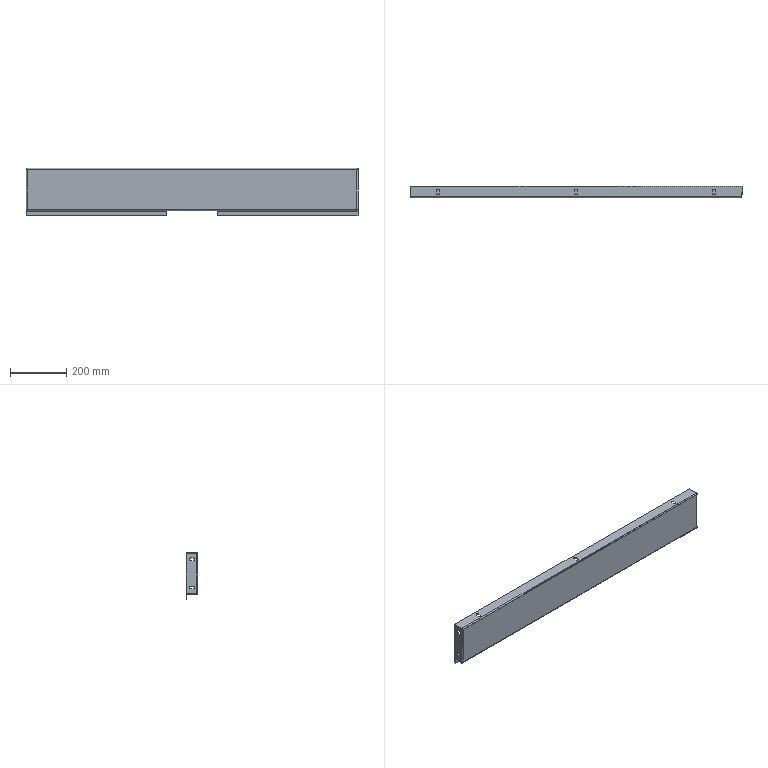Component | SolidWorks | MiddleBeam-2 | 1 solid | 98 faces | volume 577644 mm3 | plane 65 | cylinder 33 | commonest cylinder face diameters 10 x22 4 x6 8 x5 | material Plain Carbon Steel